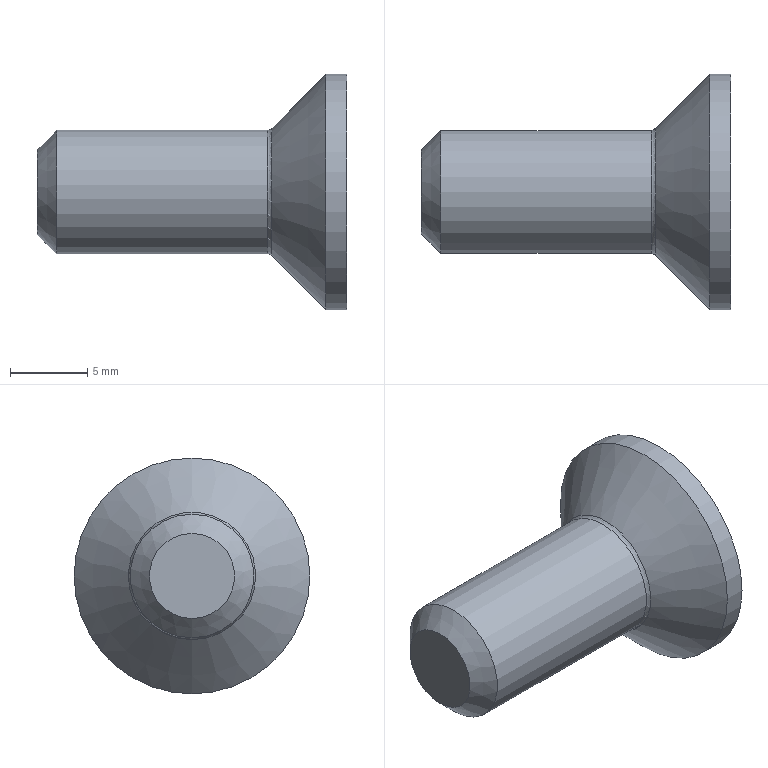Component | NX | 10_3 | 1 solid | 14 faces | volume 1300 mm3 | plane 8 | cone 3 | cylinder 2 | torus 1 | commonest cylinder face diameters 8 x1 15.24 x1